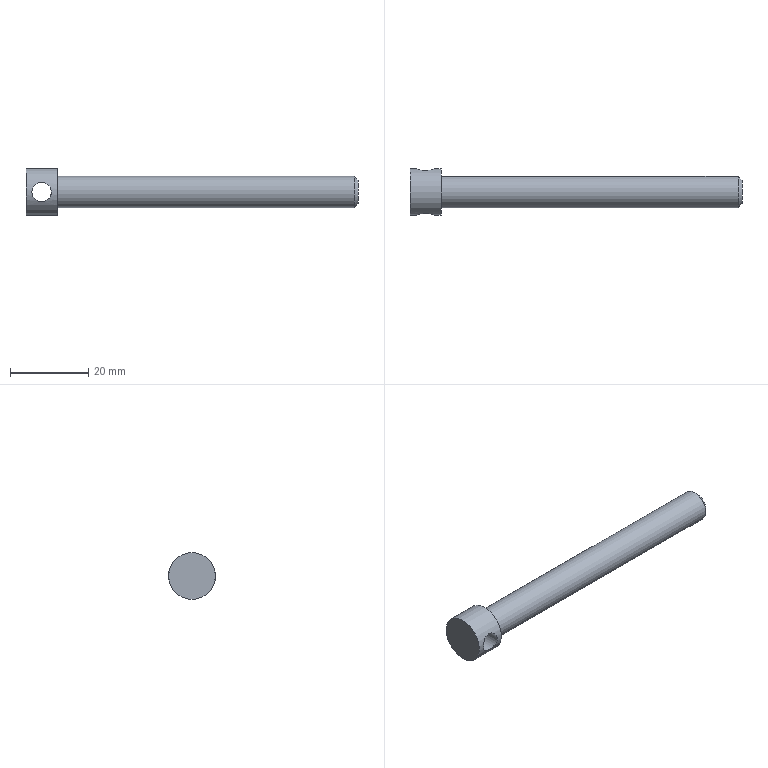Component | NX | TORQUE_SHAFT | 1 solid | 7 faces | box 85 x 12 x 12 mm | volume 4533 mm3 | cylinder 3 | plane 3 | cone 1 | commonest cylinder face diameters 12 x1 8 x1 5 x1
STEP:
#1=CARTESIAN_POINT('',(0.,0.,0.));
#2=DIRECTION('',(0.,0.,1.));
#3=DIRECTION('',(1.,0.,0.));
#4=AXIS2_PLACEMENT_3D('',#1,#2,#3);
#5=CARTESIAN_POINT('',(-16.764,70.391,12.));
#6=VERTEX_POINT('',#5);
#7=CARTESIAN_POINT('',(-16.764,70.391,18.));
#8=DIRECTION('',(-1.,0.,0.));
#9=DIRECTION('',(0.,0.,-1.));
#10=AXIS2_PLACEMENT_3D('',#7,#8,#9);
#11=CIRCLE('',#10,6.);
#12=CARTESIAN_POINT('',(-24.764,70.391,18.));
#13=DIRECTION('',(1.,0.,0.));
#14=DIRECTION('',(0.,0.,-1.));
#15=AXIS2_PLACEMENT_3D('',#12,#13,#14);
#16=CYLINDRICAL_SURFACE('',#15,6.);
#17=CARTESIAN_POINT('',(6.283,8.));
#18=DIRECTION('',(-1.,0.));
#19=VECTOR('',#18,1.);
#20=LINE('',#17,#19);
#21=(GEOMETRIC_REPRESENTATION_CONTEXT(2)PARAMETRIC_REPRESENTATION_CONTEXT()REPRESENTATION_CONTEXT('',''));
#22=DEFINITIONAL_REPRESENTATION('',(#20),#21);
#23=PCURVE('',#16,#22);
#24=CARTESIAN_POINT('',(-16.764,70.391,18.));
#25=DIRECTION('',(1.,0.,0.));
#26=DIRECTION('',(0.,0.,-1.));
#27=AXIS2_PLACEMENT_3D('',#24,#25,#26);
#28=PLANE('',#27);
#29=CARTESIAN_POINT('',(6.,0.));
#30=CARTESIAN_POINT('',(6.,-10.392));
#31=CARTESIAN_POINT('',(-3.,-5.196));
#32=CARTESIAN_POINT('',(-12.,-0.));
#33=CARTESIAN_POINT('',(-3.,5.196));
#34=CARTESIAN_POINT('',(6.,10.392));
#35=CARTESIAN_POINT('',(6.,0.));
#36=(BOUNDED_CURVE()B_SPLINE_CURVE(2,(#29,#30,#31,#32,#33,#34,#35),.UNSPECIFIED.,.T.,.F.)B_SPLINE_CURVE_WITH_KNOTS((1,2,2,2,2,1),(-2.094,0.,2.094,4.189,6.283,8.378),.UNSPECIFIED.)CURVE()GEOMETRIC_REPRESENTATION_ITEM()RATIONAL_B_SPLINE_CURVE((1.,0.5,1.,0.5,1.,0.5,1.))REPRESENTATION_ITEM(''));
#37=(GEOMETRIC_REPRESENTATION_CONTEXT(2)PARAMETRIC_REPRESENTATION_CONTEXT()REPRESENTATION_CONTEXT('',''));
#38=DEFINITIONAL_REPRESENTATION('',(#36),#37);
#39=PCURVE('',#28,#38);
#40=SURFACE_CURVE('',#11,(#23,#39),.PCURVE_S1.);
#41=EDGE_CURVE('',#6,#6,#40,.T.);
#42=ORIENTED_EDGE('',*,*,#41,.T.);
#43=CARTESIAN_POINT('',(-24.764,70.391,12.));
#44=VERTEX_POINT('',#43);
#45=CARTESIAN_POINT('',(-24.764,70.391,12.));
#46=CARTESIAN_POINT('',(-16.764,70.391,12.));
#47=B_SPLINE_CURVE_WITH_KNOTS('',1,(#45,#46),.UNSPECIFIED.,.F.,.F.,(2,2),(0.,8.),.PIECEWISE_BEZIER_KNOTS.);
#48=CARTESIAN_POINT('',(0.,0.));
#49=DIRECTION('',(0.,1.));
#50=VECTOR('',#49,1.);
#51=LINE('',#48,#50);
#52=(GEOMETRIC_REPRESENTATION_CONTEXT(2)PARAMETRIC_REPRESENTATION_CONTEXT()REPRESENTATION_CONTEXT('',''));
#53=DEFINITIONAL_REPRESENTATION('',(#51),#52);
#54=PCURVE('',#16,#53);
#55=CARTESIAN_POINT('',(6.283,0.));
#56=DIRECTION('',(0.,1.));
#57=VECTOR('',#56,1.);
#58=LINE('',#55,#57);
#59=(GEOMETRIC_REPRESENTATION_CONTEXT(2)PARAMETRIC_REPRESENTATION_CONTEXT()REPRESENTATION_CONTEXT('',''));
#60=DEFINITIONAL_REPRESENTATION('',(#58),#59);
#61=PCURVE('',#16,#60);
#62=SEAM_CURVE('',#47,(#54,#61),.PCURVE_S1.);
#63=EDGE_CURVE('',#44,#6,#62,.T.);
#64=ORIENTED_EDGE('',*,*,#63,.F.);
#65=CARTESIAN_POINT('',(-24.764,70.391,18.));
#66=DIRECTION('',(1.,0.,0.));
#67=DIRECTION('',(0.,0.,-1.));
#68=AXIS2_PLACEMENT_3D('',#65,#66,#67);
#69=CIRCLE('',#68,6.);
#70=CARTESIAN_POINT('',(0.,0.));
#71=DIRECTION('',(1.,0.));
#72=VECTOR('',#71,1.);
#73=LINE('',#70,#72);
#74=(GEOMETRIC_REPRESENTATION_CONTEXT(2)PARAMETRIC_REPRESENTATION_CONTEXT()REPRESENTATION_CONTEXT('',''));
#75=DEFINITIONAL_REPRESENTATION('',(#73),#74);
#76=PCURVE('',#16,#75);
#77=CARTESIAN_POINT('',(-24.764,70.391,18.));
#78=DIRECTION('',(-1.,0.,0.));
#79=DIRECTION('',(0.,0.,1.));
#80=AXIS2_PLACEMENT_3D('',#77,#78,#79);
#81=PLANE('',#80);
#82=CARTESIAN_POINT('',(-6.,0.));
#83=CARTESIAN_POINT('',(-6.,10.392));
#84=CARTESIAN_POINT('',(3.,5.196));
#85=CARTESIAN_POINT('',(12.,0.));
#86=CARTESIAN_POINT('',(3.,-5.196));
#87=CARTESIAN_POINT('',(-6.,-10.392));
#88=CARTESIAN_POINT('',(-6.,0.));
#89=(BOUNDED_CURVE()B_SPLINE_CURVE(2,(#82,#83,#84,#85,#86,#87,#88),.UNSPECIFIED.,.T.,.F.)B_SPLINE_CURVE_WITH_KNOTS((1,2,2,2,2,1),(-2.094,0.,2.094,4.189,6.283,8.378),.UNSPECIFIED.)CURVE()GEOMETRIC_REPRESENTATION_ITEM()RATIONAL_B_SPLINE_CURVE((1.,0.5,1.,0.5,1.,0.5,1.))REPRESENTATION_ITEM(''));
#90=(GEOMETRIC_REPRESENTATION_CONTEXT(2)PARAMETRIC_REPRESENTATION_CONTEXT()REPRESENTATION_CONTEXT('',''));
#91=DEFINITIONAL_REPRESENTATION('',(#89),#90);
#92=PCURVE('',#81,#91);
#93=SURFACE_CURVE('',#69,(#76,#92),.PCURVE_S1.);
#94=EDGE_CURVE('',#44,#44,#93,.T.);
#95=ORIENTED_EDGE('',*,*,#94,.T.);
#96=ORIENTED_EDGE('',*,*,#63,.T.);
#97=EDGE_LOOP('',(#42,#64,#95,#96));
#98=FACE_BOUND('',#97,.T.);
#99=CARTESIAN_POINT('',(-18.264,76.391,18.));
#100=VERTEX_POINT('',#99);
#101=CARTESIAN_POINT('',(-18.264,76.391,18.));
#102=CARTESIAN_POINT('',(-18.264,76.391,18.267));
#103=CARTESIAN_POINT('',(-18.308,76.373,18.538));
#104=CARTESIAN_POINT('',(-18.392,76.339,18.789));
#105=CARTESIAN_POINT('',(-18.475,76.306,19.04));
#106=CARTESIAN_POINT('',(-18.6,76.258,19.279));
#107=CARTESIAN_POINT('',(-18.755,76.204,19.489));
#108=CARTESIAN_POINT('',(-18.918,76.148,19.708));
#109=CARTESIAN_POINT('',(-19.119,76.084,19.902));
#110=CARTESIAN_POINT('',(-19.343,76.028,20.057));
#111=CARTESIAN_POINT('',(-19.579,75.968,20.22));
#112=CARTESIAN_POINT('',(-19.848,75.915,20.345));
#113=CARTESIAN_POINT('',(-20.13,75.883,20.418));
#114=CARTESIAN_POINT('',(-20.397,75.852,20.488));
#115=CARTESIAN_POINT('',(-20.683,75.839,20.514));
#116=CARTESIAN_POINT('',(-20.96,75.849,20.492));
#117=CARTESIAN_POINT('',(-21.216,75.859,20.472));
#118=CARTESIAN_POINT('',(-21.471,75.887,20.411));
#119=CARTESIAN_POINT('',(-21.706,75.927,20.316));
#120=CARTESIAN_POINT('',(-21.947,75.968,20.218));
#121=CARTESIAN_POINT('',(-22.172,76.021,20.081));
#122=CARTESIAN_POINT('',(-22.369,76.077,19.917));
#123=CARTESIAN_POINT('',(-22.582,76.137,19.738));
#124=CARTESIAN_POINT('',(-22.768,76.201,19.521));
#125=CARTESIAN_POINT('',(-22.911,76.253,19.28));
#126=CARTESIAN_POINT('',(-23.057,76.307,19.035));
#127=CARTESIAN_POINT('',(-23.164,76.35,18.757));
#128=CARTESIAN_POINT('',(-23.219,76.373,18.472));
#129=CARTESIAN_POINT('',(-23.27,76.394,18.205));
#130=CARTESIAN_POINT('',(-23.277,76.397,17.924));
#131=CARTESIAN_POINT('',(-23.24,76.381,17.655));
#132=CARTESIAN_POINT('',(-23.204,76.367,17.398));
#133=CARTESIAN_POINT('',(-23.127,76.335,17.145));
#134=CARTESIAN_POINT('',(-23.016,76.293,16.915));
#135=CARTESIAN_POINT('',(-22.902,76.249,16.677));
#136=CARTESIAN_POINT('',(-22.748,76.193,16.457));
#137=CARTESIAN_POINT('',(-22.567,76.136,16.269));
#138=CARTESIAN_POINT('',(-22.373,76.075,16.067));
#139=CARTESIAN_POINT('',(-22.142,76.012,15.896));
#140=CARTESIAN_POINT('',(-21.891,75.961,15.768));
#141=CARTESIAN_POINT('',(-21.636,75.909,15.64));
#142=CARTESIAN_POINT('',(-21.351,75.87,15.553));
#143=CARTESIAN_POINT('',(-21.064,75.854,15.518));
#144=CARTESIAN_POINT('',(-20.798,75.839,15.486));
#145=CARTESIAN_POINT('',(-20.522,75.845,15.497));
#146=CARTESIAN_POINT('',(-20.261,75.869,15.551));
#147=CARTESIAN_POINT('',(-20.011,75.892,15.602));
#148=CARTESIAN_POINT('',(-19.769,75.932,15.693));
#149=CARTESIAN_POINT('',(-19.549,75.979,15.815));
#150=CARTESIAN_POINT('',(-19.316,76.03,15.944));
#151=CARTESIAN_POINT('',(-19.104,76.09,16.112));
#152=CARTESIAN_POINT('',(-18.924,76.148,16.307));
#153=CARTESIAN_POINT('',(-18.732,76.209,16.516));
#154=CARTESIAN_POINT('',(-18.572,76.269,16.763));
#155=CARTESIAN_POINT('',(-18.461,76.312,17.028));
#156=CARTESIAN_POINT('',(-18.351,76.355,17.288));
#157=CARTESIAN_POINT('',(-18.284,76.383,17.573));
#158=CARTESIAN_POINT('',(-18.268,76.39,17.858));
#159=CARTESIAN_POINT('',(-18.265,76.391,17.906));
#160=CARTESIAN_POINT('',(-18.264,76.391,17.953));
#161=CARTESIAN_POINT('',(-18.264,76.391,18.));
#162=B_SPLINE_CURVE_WITH_KNOTS('',3,(#101,#102,#103,#104,#105,#106,#107,#108,#109,#110,#111,#112,#113,#114,#115,#116,#117,#118,#119,#120,#121,#122,#123,#124,#125,#126,#127,#128,#129,#130,#131,#132,#133,#134,#135,#136,#137,#138,#139,#140,#141,#142,#143,#144,#145,#146,#147,#148,#149,#150,#151,#152,#153,#154,#155,#156,#157,#158,#159,#160,#161),.UNSPECIFIED.,.T.,.F.,(1,3,3,3,3,3,3,3,3,3,3,3,3,3,3,3,3,3,3,3,3,3,1),(-0.008825,0.,0.05069,0.1012,0.1541,0.2097,0.2625,0.3112,0.3609,0.4149,0.4703,0.522,0.5711,0.6217,0.6761,0.7313,0.7821,0.8305,0.8818,0.937,0.9912,1.,1.051),.UNSPECIFIED.);
#163=CARTESIAN_POINT('',(1.571,6.5));
#164=CARTESIAN_POINT('',(1.581,6.5));
#165=CARTESIAN_POINT('',(1.601,6.496));
#166=CARTESIAN_POINT('',(1.631,6.476));
#167=CARTESIAN_POINT('',(1.66,6.444));
#168=CARTESIAN_POINT('',(1.69,6.399));
#169=CARTESIAN_POINT('',(1.718,6.342));
#170=CARTESIAN_POINT('',(1.746,6.273));
#171=CARTESIAN_POINT('',(1.773,6.192));
#172=CARTESIAN_POINT('',(1.799,6.101));
#173=CARTESIAN_POINT('',(1.824,6.));
#174=CARTESIAN_POINT('',(1.848,5.889));
#175=CARTESIAN_POINT('',(1.87,5.769));
#176=CARTESIAN_POINT('',(1.891,5.639));
#177=CARTESIAN_POINT('',(1.911,5.502));
#178=CARTESIAN_POINT('',(1.929,5.357));
#179=CARTESIAN_POINT('',(1.945,5.205));
#180=CARTESIAN_POINT('',(1.959,5.046));
#181=CARTESIAN_POINT('',(1.972,4.881));
#182=CARTESIAN_POINT('',(1.982,4.712));
#183=CARTESIAN_POINT('',(1.99,4.539));
#184=CARTESIAN_POINT('',(1.996,4.362));
#185=CARTESIAN_POINT('',(2.,4.182));
#186=CARTESIAN_POINT('',(2.001,4.002));
#187=CARTESIAN_POINT('',(2.,3.822));
#188=CARTESIAN_POINT('',(1.996,3.643));
#189=CARTESIAN_POINT('',(1.99,3.465));
#190=CARTESIAN_POINT('',(1.982,3.291));
#191=CARTESIAN_POINT('',(1.972,3.121));
#192=CARTESIAN_POINT('',(1.96,2.957));
#193=CARTESIAN_POINT('',(1.945,2.797));
#194=CARTESIAN_POINT('',(1.929,2.645));
#195=CARTESIAN_POINT('',(1.911,2.499));
#196=CARTESIAN_POINT('',(1.891,2.362));
#197=CARTESIAN_POINT('',(1.87,2.233));
#198=CARTESIAN_POINT('',(1.848,2.112));
#199=CARTESIAN_POINT('',(1.824,2.001));
#200=CARTESIAN_POINT('',(1.799,1.899));
#201=CARTESIAN_POINT('',(1.773,1.808));
#202=CARTESIAN_POINT('',(1.746,1.728));
#203=CARTESIAN_POINT('',(1.719,1.659));
#204=CARTESIAN_POINT('',(1.69,1.602));
#205=CARTESIAN_POINT('',(1.661,1.557));
#206=CARTESIAN_POINT('',(1.631,1.524));
#207=CARTESIAN_POINT('',(1.601,1.505));
#208=CARTESIAN_POINT('',(1.571,1.498));
#209=CARTESIAN_POINT('',(1.541,1.504));
#210=CARTESIAN_POINT('',(1.511,1.523));
#211=CARTESIAN_POINT('',(1.482,1.556));
#212=CARTESIAN_POINT('',(1.452,1.601));
#213=CARTESIAN_POINT('',(1.424,1.658));
#214=CARTESIAN_POINT('',(1.396,1.726));
#215=CARTESIAN_POINT('',(1.369,1.806));
#216=CARTESIAN_POINT('',(1.343,1.897));
#217=CARTESIAN_POINT('',(1.318,1.999));
#218=CARTESIAN_POINT('',(1.294,2.11));
#219=CARTESIAN_POINT('',(1.272,2.23));
#220=CARTESIAN_POINT('',(1.251,2.359));
#221=CARTESIAN_POINT('',(1.231,2.497));
#222=CARTESIAN_POINT('',(1.213,2.642));
#223=CARTESIAN_POINT('',(1.197,2.795));
#224=CARTESIAN_POINT('',(1.182,2.952));
#225=CARTESIAN_POINT('',(1.17,3.117));
#226=CARTESIAN_POINT('',(1.16,3.287));
#227=CARTESIAN_POINT('',(1.151,3.461));
#228=CARTESIAN_POINT('',(1.145,3.638));
#229=CARTESIAN_POINT('',(1.142,3.816));
#230=CARTESIAN_POINT('',(1.141,3.997));
#231=CARTESIAN_POINT('',(1.142,4.178));
#232=CARTESIAN_POINT('',(1.145,4.358));
#233=CARTESIAN_POINT('',(1.151,4.534));
#234=CARTESIAN_POINT('',(1.159,4.709));
#235=CARTESIAN_POINT('',(1.17,4.879));
#236=CARTESIAN_POINT('',(1.182,5.044));
#237=CARTESIAN_POINT('',(1.196,5.203));
#238=CARTESIAN_POINT('',(1.213,5.355));
#239=CARTESIAN_POINT('',(1.231,5.501));
#240=CARTESIAN_POINT('',(1.25,5.639));
#241=CARTESIAN_POINT('',(1.271,5.768));
#242=CARTESIAN_POINT('',(1.294,5.888));
#243=CARTESIAN_POINT('',(1.317,5.999));
#244=CARTESIAN_POINT('',(1.342,6.101));
#245=CARTESIAN_POINT('',(1.369,6.192));
#246=CARTESIAN_POINT('',(1.395,6.273));
#247=CARTESIAN_POINT('',(1.423,6.341));
#248=CARTESIAN_POINT('',(1.452,6.398));
#249=CARTESIAN_POINT('',(1.481,6.443));
#250=CARTESIAN_POINT('',(1.511,6.476));
#251=CARTESIAN_POINT('',(1.54,6.496));
#252=CARTESIAN_POINT('',(1.561,6.5));
#253=CARTESIAN_POINT('',(1.571,6.5));
#254=B_SPLINE_CURVE_WITH_KNOTS('',3,(#163,#164,#165,#166,#167,#168,#169,#170,#171,#172,#173,#174,#175,#176,#177,#178,#179,#180,#181,#182,#183,#184,#185,#186,#187,#188,#189,#190,#191,#192,#193,#194,#195,#196,#197,#198,#199,#200,#201,#202,#203,#204,#205,#206,#207,#208,#209,#210,#211,#212,#213,#214,#215,#216,#217,#218,#219,#220,#221,#222,#223,#224,#225,#226,#227,#228,#229,#230,#231,#232,#233,#234,#235,#236,#237,#238,#239,#240,#241,#242,#243,#244,#245,#246,#247,#248,#249,#250,#251,#252,#253),.UNSPECIFIED.,.T.,.F.,(4,1,1,1,1,1,1,1,1,1,1,1,1,1,1,1,1,1,1,1,1,1,1,1,1,1,1,1,1,1,1,1,1,1,1,1,1,1,1,1,1,1,1,1,1,1,1,1,1,1,1,1,1,1,1,1,1,1,1,1,1,1,1,1,1,1,1,1,1,1,1,1,1,1,1,1,1,1,1,1,1,1,1,1,1,1,1,1,4),(0.,0.01136,0.02273,0.03409,0.04545,0.05682,0.06818,0.07955,0.09091,0.1023,0.1136,0.125,0.1364,0.1477,0.1591,0.1705,0.1818,0.1932,0.2045,0.2159,0.2273,0.2386,0.25,0.2614,0.2727,0.2841,0.2955,0.3068,0.3182,0.3295,0.3409,0.3523,0.3636,0.375,0.3864,0.3977,0.4091,0.4205,0.4318,0.4432,0.4545,0.4659,0.4773,0.4886,0.5,0.5114,0.5227,0.5341,0.5455,0.5568,0.5682,0.5795,0.5909,0.6023,0.6136,0.625,0.6364,0.6477,0.6591,0.6705,0.6818,0.6932,0.7045,0.7159,0.7273,0.7386,0.75,0.7614,0.7727,0.7841,0.7955,0.8068,0.8182,0.8295,0.8409,0.8523,0.8636,0.875,0.8864,0.8977,0.9091,0.9205,0.9318,0.9432,0.9545,0.9659,0.9773,0.9886,1.),.QUASI_UNIFORM_KNOTS.);
#255=(GEOMETRIC_REPRESENTATION_CONTEXT(2)PARAMETRIC_REPRESENTATION_CONTEXT()REPRESENTATION_CONTEXT('',''));
#256=DEFINITIONAL_REPRESENTATION('',(#254),#255);
#257=PCURVE('',#16,#256);
#258=CARTESIAN_POINT('',(-20.764,62.391,18.));
#259=DIRECTION('',(0.,1.,0.));
#260=DIRECTION('',(1.,0.,0.));
#261=AXIS2_PLACEMENT_3D('',#258,#259,#260);
#262=CYLINDRICAL_SURFACE('',#261,2.5);
#263=CARTESIAN_POINT('',(6.283,14.));
#264=CARTESIAN_POINT('',(6.259,14.));
#265=CARTESIAN_POINT('',(6.211,13.998));
#266=CARTESIAN_POINT('',(6.139,13.99));
#267=CARTESIAN_POINT('',(6.067,13.977));
#268=CARTESIAN_POINT('',(5.995,13.958));
#269=CARTESIAN_POINT('',(5.923,13.936));
#270=CARTESIAN_POINT('',(5.852,13.909));
#271=CARTESIAN_POINT('',(5.781,13.878));
#272=CARTESIAN_POINT('',(5.709,13.845));
#273=CARTESIAN_POINT('',(5.639,13.809));
#274=CARTESIAN_POINT('',(5.568,13.772));
#275=CARTESIAN_POINT('',(5.498,13.734));
#276=CARTESIAN_POINT('',(5.427,13.695));
#277=CARTESIAN_POINT('',(5.356,13.657));
#278=CARTESIAN_POINT('',(5.286,13.62));
#279=CARTESIAN_POINT('',(5.215,13.585));
#280=CARTESIAN_POINT('',(5.144,13.553));
#281=CARTESIAN_POINT('',(5.072,13.524));
#282=CARTESIAN_POINT('',(5.001,13.5));
#283=CARTESIAN_POINT('',(4.93,13.48));
#284=CARTESIAN_POINT('',(4.858,13.466));
#285=CARTESIAN_POINT('',(4.785,13.457));
#286=CARTESIAN_POINT('',(4.713,13.454));
#287=CARTESIAN_POINT('',(4.641,13.456));
#288=CARTESIAN_POINT('',(4.569,13.465));
#289=CARTESIAN_POINT('',(4.497,13.48));
#290=CARTESIAN_POINT('',(4.425,13.5));
#291=CARTESIAN_POINT('',(4.353,13.524));
#292=CARTESIAN_POINT('',(4.282,13.553));
#293=CARTESIAN_POINT('',(4.211,13.585));
#294=CARTESIAN_POINT('',(4.14,13.62));
#295=CARTESIAN_POINT('',(4.069,13.657));
#296=CARTESIAN_POINT('',(3.999,13.695));
#297=CARTESIAN_POINT('',(3.928,13.733));
#298=CARTESIAN_POINT('',(3.857,13.772));
#299=CARTESIAN_POINT('',(3.786,13.809));
#300=CARTESIAN_POINT('',(3.716,13.845));
#301=CARTESIAN_POINT('',(3.645,13.878));
#302=CARTESIAN_POINT('',(3.574,13.908));
#303=CARTESIAN_POINT('',(3.502,13.935));
#304=CARTESIAN_POINT('',(3.431,13.958));
#305=CARTESIAN_POINT('',(3.359,13.977));
#306=CARTESIAN_POINT('',(3.287,13.99));
#307=CARTESIAN_POINT('',(3.215,13.998));
#308=CARTESIAN_POINT('',(3.143,14.001));
#309=CARTESIAN_POINT('',(3.07,13.998));
#310=CARTESIAN_POINT('',(2.998,13.99));
#311=CARTESIAN_POINT('',(2.926,13.977));
#312=CARTESIAN_POINT('',(2.854,13.959));
#313=CARTESIAN_POINT('',(2.782,13.936));
#314=CARTESIAN_POINT('',(2.711,13.909));
#315=CARTESIAN_POINT('',(2.64,13.879));
#316=CARTESIAN_POINT('',(2.569,13.845));
#317=CARTESIAN_POINT('',(2.498,13.81));
#318=CARTESIAN_POINT('',(2.427,13.772));
#319=CARTESIAN_POINT('',(2.357,13.734));
#320=CARTESIAN_POINT('',(2.286,13.695));
#321=CARTESIAN_POINT('',(2.215,13.657));
#322=CARTESIAN_POINT('',(2.144,13.62));
#323=CARTESIAN_POINT('',(2.073,13.585));
#324=CARTESIAN_POINT('',(2.003,13.553));
#325=CARTESIAN_POINT('',(1.932,13.525));
#326=CARTESIAN_POINT('',(1.86,13.5));
#327=CARTESIAN_POINT('',(1.788,13.48));
#328=CARTESIAN_POINT('',(1.716,13.465));
#329=CARTESIAN_POINT('',(1.644,13.457));
#330=CARTESIAN_POINT('',(1.572,13.454));
#331=CARTESIAN_POINT('',(1.5,13.457));
#332=CARTESIAN_POINT('',(1.427,13.465));
#333=CARTESIAN_POINT('',(1.356,13.48));
#334=CARTESIAN_POINT('',(1.284,13.499));
#335=CARTESIAN_POINT('',(1.212,13.524));
#336=CARTESIAN_POINT('',(1.14,13.553));
#337=CARTESIAN_POINT('',(1.069,13.585));
#338=CARTESIAN_POINT('',(0.9984,13.62));
#339=CARTESIAN_POINT('',(0.9275,13.657));
#340=CARTESIAN_POINT('',(0.8566,13.695));
#341=CARTESIAN_POINT('',(0.7859,13.733));
#342=CARTESIAN_POINT('',(0.7156,13.772));
#343=CARTESIAN_POINT('',(0.6449,13.809));
#344=CARTESIAN_POINT('',(0.5739,13.845));
#345=CARTESIAN_POINT('',(0.5028,13.878));
#346=CARTESIAN_POINT('',(0.4316,13.909));
#347=CARTESIAN_POINT('',(0.3606,13.935));
#348=CARTESIAN_POINT('',(0.2889,13.958));
#349=CARTESIAN_POINT('',(0.2169,13.976));
#350=CARTESIAN_POINT('',(0.1446,13.99));
#351=CARTESIAN_POINT('',(0.07286,13.998));
#352=CARTESIAN_POINT('',(0.02446,14.));
#353=CARTESIAN_POINT('',(-0.,14.));
#354=B_SPLINE_CURVE_WITH_KNOTS('',3,(#263,#264,#265,#266,#267,#268,#269,#270,#271,#272,#273,#274,#275,#276,#277,#278,#279,#280,#281,#282,#283,#284,#285,#286,#287,#288,#289,#290,#291,#292,#293,#294,#295,#296,#297,#298,#299,#300,#301,#302,#303,#304,#305,#306,#307,#308,#309,#310,#311,#312,#313,#314,#315,#316,#317,#318,#319,#320,#321,#322,#323,#324,#325,#326,#327,#328,#329,#330,#331,#332,#333,#334,#335,#336,#337,#338,#339,#340,#341,#342,#343,#344,#345,#346,#347,#348,#349,#350,#351,#352,#353),.UNSPECIFIED.,.F.,.F.,(4,1,1,1,1,1,1,1,1,1,1,1,1,1,1,1,1,1,1,1,1,1,1,1,1,1,1,1,1,1,1,1,1,1,1,1,1,1,1,1,1,1,1,1,1,1,1,1,1,1,1,1,1,1,1,1,1,1,1,1,1,1,1,1,1,1,1,1,1,1,1,1,1,1,1,1,1,1,1,1,1,1,1,1,1,1,1,1,4),(0.,0.01136,0.02273,0.03409,0.04545,0.05682,0.06818,0.07955,0.09091,0.1023,0.1136,0.125,0.1364,0.1477,0.1591,0.1705,0.1818,0.1932,0.2045,0.2159,0.2273,0.2386,0.25,0.2614,0.2727,0.2841,0.2955,0.3068,0.3182,0.3295,0.3409,0.3523,0.3636,0.375,0.3864,0.3977,0.4091,0.4205,0.4318,0.4432,0.4545,0.4659,0.4773,0.4886,0.5,0.5114,0.5227,0.5341,0.5455,0.5568,0.5682,0.5795,0.5909,0.6023,0.6136,0.625,0.6364,0.6477,0.6591,0.6705,0.6818,0.6932,0.7045,0.7159,0.7273,0.7386,0.75,0.7614,0.7727,0.7841,0.7955,0.8068,0.8182,0.8295,0.8409,0.8523,0.8636,0.875,0.8864,0.8977,0.9091,0.9205,0.9318,0.9432,0.9545,0.9659,0.9773,0.9886,1.),.QUASI_UNIFORM_KNOTS.);
#355=(GEOMETRIC_REPRESENTATION_CONTEXT(2)PARAMETRIC_REPRESENTATION_CONTEXT()REPRESENTATION_CONTEXT('',''));
#356=DEFINITIONAL_REPRESENTATION('',(#354),#355);
#357=PCURVE('',#262,#356);
#358=SURFACE_CURVE('',#162,(#257,#357),.PCURVE_S1.);
#359=EDGE_CURVE('',#100,#100,#358,.T.);
#360=ORIENTED_EDGE('',*,*,#359,.T.);
#361=EDGE_LOOP('',(#360));
#362=FACE_BOUND('',#361,.T.);
#363=CARTESIAN_POINT('',(-18.264,64.391,18.));
#364=VERTEX_POINT('',#363);
#365=CARTESIAN_POINT('',(-18.264,64.391,18.));
#366=CARTESIAN_POINT('',(-18.264,64.391,17.733));
#367=CARTESIAN_POINT('',(-18.308,64.41,17.462));
#368=CARTESIAN_POINT('',(-18.392,64.444,17.211));
#369=CARTESIAN_POINT('',(-18.475,64.477,16.96));
#370=CARTESIAN_POINT('',(-18.6,64.525,16.721));
#371=CARTESIAN_POINT('',(-18.755,64.579,16.511));
#372=CARTESIAN_POINT('',(-18.918,64.635,16.292));
#373=CARTESIAN_POINT('',(-19.119,64.699,16.098));
#374=CARTESIAN_POINT('',(-19.343,64.755,15.943));
#375=CARTESIAN_POINT('',(-19.579,64.815,15.78));
#376=CARTESIAN_POINT('',(-19.848,64.868,15.655));
#377=CARTESIAN_POINT('',(-20.13,64.9,15.582));
#378=CARTESIAN_POINT('',(-20.397,64.931,15.512));
#379=CARTESIAN_POINT('',(-20.683,64.944,15.486));
#380=CARTESIAN_POINT('',(-20.96,64.934,15.508));
#381=CARTESIAN_POINT('',(-21.216,64.924,15.528));
#382=CARTESIAN_POINT('',(-21.471,64.896,15.589));
#383=CARTESIAN_POINT('',(-21.706,64.856,15.684));
#384=CARTESIAN_POINT('',(-21.947,64.815,15.782));
#385=CARTESIAN_POINT('',(-22.172,64.761,15.919));
#386=CARTESIAN_POINT('',(-22.369,64.706,16.083));
#387=CARTESIAN_POINT('',(-22.582,64.646,16.262));
#388=CARTESIAN_POINT('',(-22.768,64.582,16.479));
#389=CARTESIAN_POINT('',(-22.911,64.53,16.72));
#390=CARTESIAN_POINT('',(-23.057,64.476,16.965));
#391=CARTESIAN_POINT('',(-23.164,64.433,17.243));
#392=CARTESIAN_POINT('',(-23.219,64.41,17.528));
#393=CARTESIAN_POINT('',(-23.27,64.389,17.795));
#394=CARTESIAN_POINT('',(-23.277,64.386,18.076));
#395=CARTESIAN_POINT('',(-23.24,64.401,18.345));
#396=CARTESIAN_POINT('',(-23.204,64.416,18.602));
#397=CARTESIAN_POINT('',(-23.127,64.448,18.855));
#398=CARTESIAN_POINT('',(-23.016,64.49,19.085));
#399=CARTESIAN_POINT('',(-22.902,64.534,19.323));
#400=CARTESIAN_POINT('',(-22.748,64.59,19.543));
#401=CARTESIAN_POINT('',(-22.567,64.647,19.731));
#402=CARTESIAN_POINT('',(-22.373,64.707,19.933));
#403=CARTESIAN_POINT('',(-22.142,64.771,20.104));
#404=CARTESIAN_POINT('',(-21.891,64.822,20.232));
#405=CARTESIAN_POINT('',(-21.636,64.873,20.36));
#406=CARTESIAN_POINT('',(-21.351,64.913,20.447));
#407=CARTESIAN_POINT('',(-21.064,64.929,20.482));
#408=CARTESIAN_POINT('',(-20.798,64.943,20.514));
#409=CARTESIAN_POINT('',(-20.522,64.938,20.503));
#410=CARTESIAN_POINT('',(-20.261,64.914,20.449));
#411=CARTESIAN_POINT('',(-20.011,64.891,20.398));
#412=CARTESIAN_POINT('',(-19.769,64.851,20.307));
#413=CARTESIAN_POINT('',(-19.549,64.803,20.185));
#414=CARTESIAN_POINT('',(-19.316,64.753,20.056));
#415=CARTESIAN_POINT('',(-19.104,64.693,19.888));
#416=CARTESIAN_POINT('',(-18.924,64.635,19.693));
#417=CARTESIAN_POINT('',(-18.732,64.574,19.484));
#418=CARTESIAN_POINT('',(-18.572,64.514,19.237));
#419=CARTESIAN_POINT('',(-18.461,64.471,18.972));
#420=CARTESIAN_POINT('',(-18.351,64.428,18.712));
#421=CARTESIAN_POINT('',(-18.284,64.4,18.427));
#422=CARTESIAN_POINT('',(-18.268,64.393,18.142));
#423=CARTESIAN_POINT('',(-18.265,64.392,18.094));
#424=CARTESIAN_POINT('',(-18.264,64.391,18.047));
#425=CARTESIAN_POINT('',(-18.264,64.391,18.));
#426=B_SPLINE_CURVE_WITH_KNOTS('',3,(#365,#366,#367,#368,#369,#370,#371,#372,#373,#374,#375,#376,#377,#378,#379,#380,#381,#382,#383,#384,#385,#386,#387,#388,#389,#390,#391,#392,#393,#394,#395,#396,#397,#398,#399,#400,#401,#402,#403,#404,#405,#406,#407,#408,#409,#410,#411,#412,#413,#414,#415,#416,#417,#418,#419,#420,#421,#422,#423,#424,#425),.UNSPECIFIED.,.T.,.F.,(1,3,3,3,3,3,3,3,3,3,3,3,3,3,3,3,3,3,3,3,3,3,1),(-0.008825,0.,0.05069,0.1012,0.1541,0.2097,0.2625,0.3112,0.3609,0.4149,0.4703,0.522,0.5711,0.6217,0.6761,0.7313,0.7821,0.8305,0.8818,0.937,0.9912,1.,1.051),.UNSPECIFIED.);
#427=CARTESIAN_POINT('',(4.712,6.5));
#428=CARTESIAN_POINT('',(4.722,6.5));
#429=CARTESIAN_POINT('',(4.742,6.496));
#430=CARTESIAN_POINT('',(4.772,6.476));
#431=CARTESIAN_POINT('',(4.802,6.444));
#432=CARTESIAN_POINT('',(4.831,6.399));
#433=CARTESIAN_POINT('',(4.86,6.342));
#434=CARTESIAN_POINT('',(4.888,6.273));
#435=CARTESIAN_POINT('',(4.915,6.192));
#436=CARTESIAN_POINT('',(4.941,6.101));
#437=CARTESIAN_POINT('',(4.966,6.));
#438=CARTESIAN_POINT('',(4.989,5.889));
#439=CARTESIAN_POINT('',(5.012,5.769));
#440=CARTESIAN_POINT('',(5.033,5.639));
#441=CARTESIAN_POINT('',(5.052,5.502));
#442=CARTESIAN_POINT('',(5.07,5.357));
#443=CARTESIAN_POINT('',(5.086,5.205));
#444=CARTESIAN_POINT('',(5.101,5.046));
#445=CARTESIAN_POINT('',(5.113,4.881));
#446=CARTESIAN_POINT('',(5.124,4.712));
#447=CARTESIAN_POINT('',(5.132,4.539));
#448=CARTESIAN_POINT('',(5.138,4.362));
#449=CARTESIAN_POINT('',(5.141,4.182));
#450=CARTESIAN_POINT('',(5.143,4.002));
#451=CARTESIAN_POINT('',(5.141,3.822));
#452=CARTESIAN_POINT('',(5.138,3.643));
#453=CARTESIAN_POINT('',(5.132,3.465));
#454=CARTESIAN_POINT('',(5.124,3.291));
#455=CARTESIAN_POINT('',(5.113,3.121));
#456=CARTESIAN_POINT('',(5.101,2.957));
#457=CARTESIAN_POINT('',(5.087,2.797));
#458=CARTESIAN_POINT('',(5.07,2.645));
#459=CARTESIAN_POINT('',(5.053,2.499));
#460=CARTESIAN_POINT('',(5.033,2.362));
#461=CARTESIAN_POINT('',(5.012,2.233));
#462=CARTESIAN_POINT('',(4.99,2.112));
#463=CARTESIAN_POINT('',(4.966,2.001));
#464=CARTESIAN_POINT('',(4.941,1.899));
#465=CARTESIAN_POINT('',(4.915,1.808));
#466=CARTESIAN_POINT('',(4.888,1.728));
#467=CARTESIAN_POINT('',(4.86,1.659));
#468=CARTESIAN_POINT('',(4.832,1.602));
#469=CARTESIAN_POINT('',(4.802,1.557));
#470=CARTESIAN_POINT('',(4.773,1.524));
#471=CARTESIAN_POINT('',(4.743,1.505));
#472=CARTESIAN_POINT('',(4.713,1.498));
#473=CARTESIAN_POINT('',(4.683,1.504));
#474=CARTESIAN_POINT('',(4.653,1.523));
#475=CARTESIAN_POINT('',(4.623,1.556));
#476=CARTESIAN_POINT('',(4.594,1.601));
#477=CARTESIAN_POINT('',(4.565,1.658));
#478=CARTESIAN_POINT('',(4.537,1.726));
#479=CARTESIAN_POINT('',(4.511,1.806));
#480=CARTESIAN_POINT('',(4.484,1.897));
#481=CARTESIAN_POINT('',(4.459,1.999));
#482=CARTESIAN_POINT('',(4.436,2.11));
#483=CARTESIAN_POINT('',(4.413,2.23));
#484=CARTESIAN_POINT('',(4.392,2.359));
#485=CARTESIAN_POINT('',(4.373,2.497));
#486=CARTESIAN_POINT('',(4.355,2.642));
#487=CARTESIAN_POINT('',(4.338,2.795));
#488=CARTESIAN_POINT('',(4.324,2.952));
#489=CARTESIAN_POINT('',(4.312,3.117));
#490=CARTESIAN_POINT('',(4.301,3.287));
#491=CARTESIAN_POINT('',(4.293,3.461));
#492=CARTESIAN_POINT('',(4.287,3.638));
#493=CARTESIAN_POINT('',(4.283,3.816));
#494=CARTESIAN_POINT('',(4.282,3.997));
#495=CARTESIAN_POINT('',(4.283,4.178));
#496=CARTESIAN_POINT('',(4.287,4.358));
#497=CARTESIAN_POINT('',(4.293,4.534));
#498=CARTESIAN_POINT('',(4.301,4.709));
#499=CARTESIAN_POINT('',(4.311,4.879));
#500=CARTESIAN_POINT('',(4.324,5.044));
#501=CARTESIAN_POINT('',(4.338,5.203));
#502=CARTESIAN_POINT('',(4.354,5.355));
#503=CARTESIAN_POINT('',(4.372,5.501));
#504=CARTESIAN_POINT('',(4.392,5.639));
#505=CARTESIAN_POINT('',(4.413,5.768));
#506=CARTESIAN_POINT('',(4.435,5.888));
#507=CARTESIAN_POINT('',(4.459,5.999));
#508=CARTESIAN_POINT('',(4.484,6.101));
#509=CARTESIAN_POINT('',(4.51,6.192));
#510=CARTESIAN_POINT('',(4.537,6.273));
#511=CARTESIAN_POINT('',(4.565,6.341));
#512=CARTESIAN_POINT('',(4.593,6.398));
#513=CARTESIAN_POINT('',(4.623,6.443));
#514=CARTESIAN_POINT('',(4.652,6.476));
#515=CARTESIAN_POINT('',(4.682,6.496));
#516=CARTESIAN_POINT('',(4.702,6.5));
#517=CARTESIAN_POINT('',(4.712,6.5));
#518=B_SPLINE_CURVE_WITH_KNOTS('',3,(#427,#428,#429,#430,#431,#432,#433,#434,#435,#436,#437,#438,#439,#440,#441,#442,#443,#444,#445,#446,#447,#448,#449,#450,#451,#452,#453,#454,#455,#456,#457,#458,#459,#460,#461,#462,#463,#464,#465,#466,#467,#468,#469,#470,#471,#472,#473,#474,#475,#476,#477,#478,#479,#480,#481,#482,#483,#484,#485,#486,#487,#488,#489,#490,#491,#492,#493,#494,#495,#496,#497,#498,#499,#500,#501,#502,#503,#504,#505,#506,#507,#508,#509,#510,#511,#512,#513,#514,#515,#516,#517),.UNSPECIFIED.,.T.,.F.,(4,1,1,1,1,1,1,1,1,1,1,1,1,1,1,1,1,1,1,1,1,1,1,1,1,1,1,1,1,1,1,1,1,1,1,1,1,1,1,1,1,1,1,1,1,1,1,1,1,1,1,1,1,1,1,1,1,1,1,1,1,1,1,1,1,1,1,1,1,1,1,1,1,1,1,1,1,1,1,1,1,1,1,1,1,1,1,1,4),(0.,0.01136,0.02273,0.03409,0.04545,0.05682,0.06818,0.07955,0.09091,0.1023,0.1136,0.125,0.1364,0.1477,0.1591,0.1705,0.1818,0.1932,0.2045,0.2159,0.2273,0.2386,0.25,0.2614,0.2727,0.2841,0.2955,0.3068,0.3182,0.3295,0.3409,0.3523,0.3636,0.375,0.3864,0.3977,0.4091,0.4205,0.4318,0.4432,0.4545,0.4659,0.4773,0.4886,0.5,0.5114,0.5227,0.5341,0.5455,0.5568,0.5682,0.5795,0.5909,0.6023,0.6136,0.625,0.6364,0.6477,0.6591,0.6705,0.6818,0.6932,0.7045,0.7159,0.7273,0.7386,0.75,0.7614,0.7727,0.7841,0.7955,0.8068,0.8182,0.8295,0.8409,0.8523,0.8636,0.875,0.8864,0.8977,0.9091,0.9205,0.9318,0.9432,0.9545,0.9659,0.9773,0.9886,1.),.QUASI_UNIFORM_KNOTS.);
#519=(GEOMETRIC_REPRESENTATION_CONTEXT(2)PARAMETRIC_REPRESENTATION_CONTEXT()REPRESENTATION_CONTEXT('',''));
#520=DEFINITIONAL_REPRESENTATION('',(#518),#519);
#521=PCURVE('',#16,#520);
#522=CARTESIAN_POINT('',(0.,2.));
#523=CARTESIAN_POINT('',(0.02395,2.));
#524=CARTESIAN_POINT('',(0.07201,2.002));
#525=CARTESIAN_POINT('',(0.1443,2.01));
#526=CARTESIAN_POINT('',(0.2165,2.023));
#527=CARTESIAN_POINT('',(0.2884,2.042));
#528=CARTESIAN_POINT('',(0.3597,2.064));
#529=CARTESIAN_POINT('',(0.4312,2.091));
#530=CARTESIAN_POINT('',(0.5026,2.122));
#531=CARTESIAN_POINT('',(0.5738,2.155));
#532=CARTESIAN_POINT('',(0.6444,2.191));
#533=CARTESIAN_POINT('',(0.7149,2.228));
#534=CARTESIAN_POINT('',(0.7857,2.266));
#535=CARTESIAN_POINT('',(0.8564,2.305));
#536=CARTESIAN_POINT('',(0.9271,2.343));
#537=CARTESIAN_POINT('',(0.9974,2.38));
#538=CARTESIAN_POINT('',(1.068,2.415));
#539=CARTESIAN_POINT('',(1.139,2.447));
#540=CARTESIAN_POINT('',(1.211,2.476));
#541=CARTESIAN_POINT('',(1.282,2.5));
#542=CARTESIAN_POINT('',(1.354,2.52));
#543=CARTESIAN_POINT('',(1.426,2.534));
#544=CARTESIAN_POINT('',(1.498,2.543));
#545=CARTESIAN_POINT('',(1.57,2.546));
#546=CARTESIAN_POINT('',(1.642,2.544));
#547=CARTESIAN_POINT('',(1.714,2.535));
#548=CARTESIAN_POINT('',(1.786,2.52));
#549=CARTESIAN_POINT('',(1.858,2.5));
#550=CARTESIAN_POINT('',(1.93,2.476));
#551=CARTESIAN_POINT('',(2.001,2.447));
#552=CARTESIAN_POINT('',(2.072,2.415));
#553=CARTESIAN_POINT('',(2.143,2.38));
#554=CARTESIAN_POINT('',(2.214,2.343));
#555=CARTESIAN_POINT('',(2.285,2.305));
#556=CARTESIAN_POINT('',(2.355,2.267));
#557=CARTESIAN_POINT('',(2.426,2.228));
#558=CARTESIAN_POINT('',(2.497,2.191));
#559=CARTESIAN_POINT('',(2.568,2.155));
#560=CARTESIAN_POINT('',(2.638,2.122));
#561=CARTESIAN_POINT('',(2.709,2.092));
#562=CARTESIAN_POINT('',(2.781,2.065));
#563=CARTESIAN_POINT('',(2.853,2.042));
#564=CARTESIAN_POINT('',(2.924,2.023));
#565=CARTESIAN_POINT('',(2.996,2.01));
#566=CARTESIAN_POINT('',(3.068,2.002));
#567=CARTESIAN_POINT('',(3.141,1.999));
#568=CARTESIAN_POINT('',(3.213,2.002));
#569=CARTESIAN_POINT('',(3.285,2.01));
#570=CARTESIAN_POINT('',(3.357,2.023));
#571=CARTESIAN_POINT('',(3.429,2.041));
#572=CARTESIAN_POINT('',(3.501,2.064));
#573=CARTESIAN_POINT('',(3.572,2.091));
#574=CARTESIAN_POINT('',(3.643,2.121));
#575=CARTESIAN_POINT('',(3.714,2.155));
#576=CARTESIAN_POINT('',(3.785,2.19));
#577=CARTESIAN_POINT('',(3.856,2.228));
#578=CARTESIAN_POINT('',(3.927,2.266));
#579=CARTESIAN_POINT('',(3.997,2.305));
#580=CARTESIAN_POINT('',(4.068,2.343));
#581=CARTESIAN_POINT('',(4.139,2.38));
#582=CARTESIAN_POINT('',(4.21,2.415));
#583=CARTESIAN_POINT('',(4.28,2.447));
#584=CARTESIAN_POINT('',(4.352,2.475));
#585=CARTESIAN_POINT('',(4.423,2.5));
#586=CARTESIAN_POINT('',(4.495,2.52));
#587=CARTESIAN_POINT('',(4.567,2.535));
#588=CARTESIAN_POINT('',(4.639,2.543));
#589=CARTESIAN_POINT('',(4.711,2.546));
#590=CARTESIAN_POINT('',(4.784,2.543));
#591=CARTESIAN_POINT('',(4.856,2.535));
#592=CARTESIAN_POINT('',(4.928,2.52));
#593=CARTESIAN_POINT('',(4.999,2.501));
#594=CARTESIAN_POINT('',(5.071,2.476));
#595=CARTESIAN_POINT('',(5.143,2.447));
#596=CARTESIAN_POINT('',(5.214,2.415));
#597=CARTESIAN_POINT('',(5.285,2.38));
#598=CARTESIAN_POINT('',(5.356,2.343));
#599=CARTESIAN_POINT('',(5.427,2.305));
#600=CARTESIAN_POINT('',(5.497,2.267));
#601=CARTESIAN_POINT('',(5.568,2.228));
#602=CARTESIAN_POINT('',(5.638,2.191));
#603=CARTESIAN_POINT('',(5.709,2.155));
#604=CARTESIAN_POINT('',(5.78,2.122));
#605=CARTESIAN_POINT('',(5.852,2.091));
#606=CARTESIAN_POINT('',(5.923,2.065));
#607=CARTESIAN_POINT('',(5.994,2.042));
#608=CARTESIAN_POINT('',(6.066,2.024));
#609=CARTESIAN_POINT('',(6.139,2.01));
#610=CARTESIAN_POINT('',(6.21,2.002));
#611=CARTESIAN_POINT('',(6.259,2.));
#612=CARTESIAN_POINT('',(6.283,2.));
#613=B_SPLINE_CURVE_WITH_KNOTS('',3,(#522,#523,#524,#525,#526,#527,#528,#529,#530,#531,#532,#533,#534,#535,#536,#537,#538,#539,#540,#541,#542,#543,#544,#545,#546,#547,#548,#549,#550,#551,#552,#553,#554,#555,#556,#557,#558,#559,#560,#561,#562,#563,#564,#565,#566,#567,#568,#569,#570,#571,#572,#573,#574,#575,#576,#577,#578,#579,#580,#581,#582,#583,#584,#585,#586,#587,#588,#589,#590,#591,#592,#593,#594,#595,#596,#597,#598,#599,#600,#601,#602,#603,#604,#605,#606,#607,#608,#609,#610,#611,#612),.UNSPECIFIED.,.F.,.F.,(4,1,1,1,1,1,1,1,1,1,1,1,1,1,1,1,1,1,1,1,1,1,1,1,1,1,1,1,1,1,1,1,1,1,1,1,1,1,1,1,1,1,1,1,1,1,1,1,1,1,1,1,1,1,1,1,1,1,1,1,1,1,1,1,1,1,1,1,1,1,1,1,1,1,1,1,1,1,1,1,1,1,1,1,1,1,1,1,4),(0.,0.01136,0.02273,0.03409,0.04545,0.05682,0.06818,0.07955,0.09091,0.1023,0.1136,0.125,0.1364,0.1477,0.1591,0.1705,0.1818,0.1932,0.2045,0.2159,0.2273,0.2386,0.25,0.2614,0.2727,0.2841,0.2955,0.3068,0.3182,0.3295,0.3409,0.3523,0.3636,0.375,0.3864,0.3977,0.4091,0.4205,0.4318,0.4432,0.4545,0.4659,0.4773,0.4886,0.5,0.5114,0.5227,0.5341,0.5455,0.5568,0.5682,0.5795,0.5909,0.6023,0.6136,0.625,0.6364,0.6477,0.6591,0.6705,0.6818,0.6932,0.7045,0.7159,0.7273,0.7386,0.75,0.7614,0.7727,0.7841,0.7955,0.8068,0.8182,0.8295,0.8409,0.8523,0.8636,0.875,0.8864,0.8977,0.9091,0.9205,0.9318,0.9432,0.9545,0.9659,0.9773,0.9886,1.),.QUASI_UNIFORM_KNOTS.);
#614=(GEOMETRIC_REPRESENTATION_CONTEXT(2)PARAMETRIC_REPRESENTATION_CONTEXT()REPRESENTATION_CONTEXT('',''));
#615=DEFINITIONAL_REPRESENTATION('',(#613),#614);
#616=PCURVE('',#262,#615);
#617=SURFACE_CURVE('',#426,(#521,#616),.PCURVE_S1.);
#618=EDGE_CURVE('',#364,#364,#617,.T.);
#619=ORIENTED_EDGE('',*,*,#618,.T.);
#620=EDGE_LOOP('',(#619));
#621=FACE_BOUND('',#620,.T.);
#622=ADVANCED_FACE('',(#98,#362,#621),#16,.T.);
#623=CARTESIAN_POINT('',(59.236,70.391,22.));
#624=VERTEX_POINT('',#623);
#625=CARTESIAN_POINT('',(59.236,70.391,14.));
#626=VERTEX_POINT('',#625);
#627=CARTESIAN_POINT('',(59.236,70.391,18.));
#628=DIRECTION('',(-1.,0.,0.));
#629=DIRECTION('',(0.,0.,1.));
#630=AXIS2_PLACEMENT_3D('',#627,#628,#629);
#631=CIRCLE('',#630,4.);
#632=CARTESIAN_POINT('',(-24.764,70.391,18.));
#633=DIRECTION('',(1.,0.,0.));
#634=DIRECTION('',(0.,0.,-1.));
#635=AXIS2_PLACEMENT_3D('',#632,#633,#634);
#636=CYLINDRICAL_SURFACE('',#635,4.);
#637=CARTESIAN_POINT('',(3.142,84.));
#638=DIRECTION('',(-1.,0.));
#639=VECTOR('',#638,1.);
#640=LINE('',#637,#639);
#641=(GEOMETRIC_REPRESENTATION_CONTEXT(2)PARAMETRIC_REPRESENTATION_CONTEXT()REPRESENTATION_CONTEXT('',''));
#642=DEFINITIONAL_REPRESENTATION('',(#640),#641);
#643=PCURVE('',#636,#642);
#644=CARTESIAN_POINT('',(59.236,70.391,18.));
#645=DIRECTION('',(-1.,0.,0.));
#646=DIRECTION('',(0.,0.,1.));
#647=AXIS2_PLACEMENT_3D('',#644,#645,#646);
#648=CONICAL_SURFACE('',#647,4.,0.7854);
#649=CARTESIAN_POINT('',(0.,0.));
#650=DIRECTION('',(1.,0.));
#651=VECTOR('',#650,1.);
#652=LINE('',#649,#651);
#653=(GEOMETRIC_REPRESENTATION_CONTEXT(2)PARAMETRIC_REPRESENTATION_CONTEXT()REPRESENTATION_CONTEXT('',''));
#654=DEFINITIONAL_REPRESENTATION('',(#652),#653);
#655=PCURVE('',#648,#654);
#656=SURFACE_CURVE('',#631,(#643,#655),.PCURVE_S1.);
#657=EDGE_CURVE('',#624,#626,#656,.T.);
#658=ORIENTED_EDGE('',*,*,#657,.T.);
#659=CARTESIAN_POINT('',(-16.764,70.391,14.));
#660=VERTEX_POINT('',#659);
#661=CARTESIAN_POINT('',(-16.764,70.391,14.));
#662=CARTESIAN_POINT('',(59.236,70.391,14.));
#663=B_SPLINE_CURVE_WITH_KNOTS('',1,(#661,#662),.UNSPECIFIED.,.F.,.F.,(2,2),(8.,84.),.PIECEWISE_BEZIER_KNOTS.);
#664=CARTESIAN_POINT('',(0.,0.));
#665=DIRECTION('',(0.,1.));
#666=VECTOR('',#665,1.);
#667=LINE('',#664,#666);
#668=(GEOMETRIC_REPRESENTATION_CONTEXT(2)PARAMETRIC_REPRESENTATION_CONTEXT()REPRESENTATION_CONTEXT('',''));
#669=DEFINITIONAL_REPRESENTATION('',(#667),#668);
#670=PCURVE('',#636,#669);
#671=CARTESIAN_POINT('',(6.283,0.));
#672=DIRECTION('',(0.,1.));
#673=VECTOR('',#672,1.);
#674=LINE('',#671,#673);
#675=(GEOMETRIC_REPRESENTATION_CONTEXT(2)PARAMETRIC_REPRESENTATION_CONTEXT()REPRESENTATION_CONTEXT('',''));
#676=DEFINITIONAL_REPRESENTATION('',(#674),#675);
#677=PCURVE('',#636,#676);
#678=SEAM_CURVE('',#663,(#670,#677),.PCURVE_S1.);
#679=EDGE_CURVE('',#660,#626,#678,.T.);
#680=ORIENTED_EDGE('',*,*,#679,.F.);
#681=CARTESIAN_POINT('',(-16.764,70.391,18.));
#682=DIRECTION('',(-1.,0.,0.));
#683=DIRECTION('',(0.,0.,-1.));
#684=AXIS2_PLACEMENT_3D('',#681,#682,#683);
#685=CIRCLE('',#684,4.);
#686=CARTESIAN_POINT('',(6.283,8.));
#687=DIRECTION('',(-1.,0.));
#688=VECTOR('',#687,1.);
#689=LINE('',#686,#688);
#690=(GEOMETRIC_REPRESENTATION_CONTEXT(2)PARAMETRIC_REPRESENTATION_CONTEXT()REPRESENTATION_CONTEXT('',''));
#691=DEFINITIONAL_REPRESENTATION('',(#689),#690);
#692=PCURVE('',#636,#691);
#693=CARTESIAN_POINT('',(4.,0.));
#694=CARTESIAN_POINT('',(4.,-6.928));
#695=CARTESIAN_POINT('',(-2.,-3.464));
#696=CARTESIAN_POINT('',(-8.,-0.));
#697=CARTESIAN_POINT('',(-2.,3.464));
#698=CARTESIAN_POINT('',(4.,6.928));
#699=CARTESIAN_POINT('',(4.,0.));
#700=(BOUNDED_CURVE()B_SPLINE_CURVE(2,(#693,#694,#695,#696,#697,#698,#699),.UNSPECIFIED.,.T.,.F.)B_SPLINE_CURVE_WITH_KNOTS((1,2,2,2,2,1),(-2.094,0.,2.094,4.189,6.283,8.378),.UNSPECIFIED.)CURVE()GEOMETRIC_REPRESENTATION_ITEM()RATIONAL_B_SPLINE_CURVE((1.,0.5,1.,0.5,1.,0.5,1.))REPRESENTATION_ITEM(''));
#701=(GEOMETRIC_REPRESENTATION_CONTEXT(2)PARAMETRIC_REPRESENTATION_CONTEXT()REPRESENTATION_CONTEXT('',''));
#702=DEFINITIONAL_REPRESENTATION('',(#700),#701);
#703=PCURVE('',#28,#702);
#704=SURFACE_CURVE('',#685,(#692,#703),.PCURVE_S1.);
#705=EDGE_CURVE('',#660,#660,#704,.T.);
#706=ORIENTED_EDGE('',*,*,#705,.F.);
#707=ORIENTED_EDGE('',*,*,#679,.T.);
#708=CARTESIAN_POINT('',(59.236,70.391,18.));
#709=DIRECTION('',(-1.,0.,0.));
#710=DIRECTION('',(0.,0.,1.));
#711=AXIS2_PLACEMENT_3D('',#708,#709,#710);
#712=CIRCLE('',#711,4.);
#713=CARTESIAN_POINT('',(9.425,84.));
#714=DIRECTION('',(-1.,0.));
#715=VECTOR('',#714,1.);
#716=LINE('',#713,#715);
#717=(GEOMETRIC_REPRESENTATION_CONTEXT(2)PARAMETRIC_REPRESENTATION_CONTEXT()REPRESENTATION_CONTEXT('',''));
#718=DEFINITIONAL_REPRESENTATION('',(#716),#717);
#719=PCURVE('',#636,#718);
#720=CARTESIAN_POINT('',(0.,0.));
#721=DIRECTION('',(1.,0.));
#722=VECTOR('',#721,1.);
#723=LINE('',#720,#722);
#724=(GEOMETRIC_REPRESENTATION_CONTEXT(2)PARAMETRIC_REPRESENTATION_CONTEXT()REPRESENTATION_CONTEXT('',''));
#725=DEFINITIONAL_REPRESENTATION('',(#723),#724);
#726=PCURVE('',#648,#725);
#727=SURFACE_CURVE('',#712,(#719,#726),.PCURVE_S1.);
#728=EDGE_CURVE('',#626,#624,#727,.T.);
#729=ORIENTED_EDGE('',*,*,#728,.T.);
#730=EDGE_LOOP('',(#658,#680,#706,#707,#729));
#731=FACE_BOUND('',#730,.T.);
#732=ADVANCED_FACE('',(#731),#636,.T.);
#733=ORIENTED_EDGE('',*,*,#705,.T.);
#734=EDGE_LOOP('',(#733));
#735=FACE_BOUND('',#734,.T.);
#736=ORIENTED_EDGE('',*,*,#41,.F.);
#737=EDGE_LOOP('',(#736));
#738=FACE_BOUND('',#737,.T.);
#739=ADVANCED_FACE('',(#735,#738),#28,.T.);
#740=ORIENTED_EDGE('',*,*,#94,.F.);
#741=EDGE_LOOP('',(#740));
#742=FACE_BOUND('',#741,.T.);
#743=ADVANCED_FACE('',(#742),#81,.T.);
#744=ORIENTED_EDGE('',*,*,#618,.T.);
#745=CARTESIAN_POINT('',(-18.264,64.391,18.));
#746=CARTESIAN_POINT('',(-18.264,76.391,18.));
#747=B_SPLINE_CURVE_WITH_KNOTS('',1,(#745,#746),.UNSPECIFIED.,.F.,.F.,(2,2),(2.,14.),.PIECEWISE_BEZIER_KNOTS.);
#748=CARTESIAN_POINT('',(6.283,0.));
#749=DIRECTION('',(0.,1.));
#750=VECTOR('',#749,1.);
#751=LINE('',#748,#750);
#752=(GEOMETRIC_REPRESENTATION_CONTEXT(2)PARAMETRIC_REPRESENTATION_CONTEXT()REPRESENTATION_CONTEXT('',''));
#753=DEFINITIONAL_REPRESENTATION('',(#751),#752);
#754=PCURVE('',#262,#753);
#755=CARTESIAN_POINT('',(0.,0.));
#756=DIRECTION('',(0.,1.));
#757=VECTOR('',#756,1.);
#758=LINE('',#755,#757);
#759=(GEOMETRIC_REPRESENTATION_CONTEXT(2)PARAMETRIC_REPRESENTATION_CONTEXT()REPRESENTATION_CONTEXT('',''));
#760=DEFINITIONAL_REPRESENTATION('',(#758),#759);
#761=PCURVE('',#262,#760);
#762=SEAM_CURVE('',#747,(#754,#761),.PCURVE_S1.);
#763=EDGE_CURVE('',#364,#100,#762,.T.);
#764=ORIENTED_EDGE('',*,*,#763,.T.);
#765=ORIENTED_EDGE('',*,*,#359,.T.);
#766=ORIENTED_EDGE('',*,*,#763,.F.);
#767=EDGE_LOOP('',(#744,#764,#765,#766));
#768=FACE_BOUND('',#767,.F.);
#769=ADVANCED_FACE('',(#768),#262,.F.);
#770=CARTESIAN_POINT('',(60.236,70.391,21.));
#771=VERTEX_POINT('',#770);
#772=CARTESIAN_POINT('',(60.236,70.391,18.));
#773=DIRECTION('',(1.,0.,0.));
#774=DIRECTION('',(0.,0.,1.));
#775=AXIS2_PLACEMENT_3D('',#772,#773,#774);
#776=CIRCLE('',#775,3.);
#777=CARTESIAN_POINT('',(60.236,70.391,18.));
#778=DIRECTION('',(-1.,0.,0.));
#779=DIRECTION('',(0.,0.,1.));
#780=AXIS2_PLACEMENT_3D('',#777,#778,#779);
#781=PLANE('',#780);
#782=CARTESIAN_POINT('',(3.,0.));
#783=CARTESIAN_POINT('',(3.,-5.196));
#784=CARTESIAN_POINT('',(-1.5,-2.598));
#785=CARTESIAN_POINT('',(-6.,-0.));
#786=CARTESIAN_POINT('',(-1.5,2.598));
#787=CARTESIAN_POINT('',(3.,5.196));
#788=CARTESIAN_POINT('',(3.,0.));
#789=(BOUNDED_CURVE()B_SPLINE_CURVE(2,(#782,#783,#784,#785,#786,#787,#788),.UNSPECIFIED.,.T.,.F.)B_SPLINE_CURVE_WITH_KNOTS((1,2,2,2,2,1),(-2.094,0.,2.094,4.189,6.283,8.378),.UNSPECIFIED.)CURVE()GEOMETRIC_REPRESENTATION_ITEM()RATIONAL_B_SPLINE_CURVE((1.,0.5,1.,0.5,1.,0.5,1.))REPRESENTATION_ITEM(''));
#790=(GEOMETRIC_REPRESENTATION_CONTEXT(2)PARAMETRIC_REPRESENTATION_CONTEXT()REPRESENTATION_CONTEXT('',''));
#791=DEFINITIONAL_REPRESENTATION('',(#789),#790);
#792=PCURVE('',#781,#791);
#793=CARTESIAN_POINT('',(6.283,-1.));
#794=DIRECTION('',(-1.,0.));
#795=VECTOR('',#794,1.);
#796=LINE('',#793,#795);
#797=(GEOMETRIC_REPRESENTATION_CONTEXT(2)PARAMETRIC_REPRESENTATION_CONTEXT()REPRESENTATION_CONTEXT('',''));
#798=DEFINITIONAL_REPRESENTATION('',(#796),#797);
#799=PCURVE('',#648,#798);
#800=SURFACE_CURVE('',#776,(#792,#799),.PCURVE_S1.);
#801=EDGE_CURVE('',#771,#771,#800,.T.);
#802=ORIENTED_EDGE('',*,*,#801,.T.);
#803=EDGE_LOOP('',(#802));
#804=FACE_BOUND('',#803,.T.);
#805=ADVANCED_FACE('',(#804),#781,.F.);
#806=ORIENTED_EDGE('',*,*,#801,.F.);
#807=CARTESIAN_POINT('',(60.236,70.391,21.));
#808=CARTESIAN_POINT('',(59.236,70.391,22.));
#809=B_SPLINE_CURVE_WITH_KNOTS('',1,(#807,#808),.UNSPECIFIED.,.F.,.F.,(2,2),(-1.414,0.),.PIECEWISE_BEZIER_KNOTS.);
#810=CARTESIAN_POINT('',(6.283,0.));
#811=DIRECTION('',(0.,1.));
#812=VECTOR('',#811,1.);
#813=LINE('',#810,#812);
#814=(GEOMETRIC_REPRESENTATION_CONTEXT(2)PARAMETRIC_REPRESENTATION_CONTEXT()REPRESENTATION_CONTEXT('',''));
#815=DEFINITIONAL_REPRESENTATION('',(#813),#814);
#816=PCURVE('',#648,#815);
#817=CARTESIAN_POINT('',(0.,0.));
#818=DIRECTION('',(0.,1.));
#819=VECTOR('',#818,1.);
#820=LINE('',#817,#819);
#821=(GEOMETRIC_REPRESENTATION_CONTEXT(2)PARAMETRIC_REPRESENTATION_CONTEXT()REPRESENTATION_CONTEXT('',''));
#822=DEFINITIONAL_REPRESENTATION('',(#820),#821);
#823=PCURVE('',#648,#822);
#824=SEAM_CURVE('',#809,(#816,#823),.PCURVE_S1.);
#825=EDGE_CURVE('',#771,#624,#824,.T.);
#826=ORIENTED_EDGE('',*,*,#825,.T.);
#827=ORIENTED_EDGE('',*,*,#728,.F.);
#828=ORIENTED_EDGE('',*,*,#657,.F.);
#829=ORIENTED_EDGE('',*,*,#825,.F.);
#830=EDGE_LOOP('',(#806,#826,#827,#828,#829));
#831=FACE_BOUND('',#830,.T.);
#832=ADVANCED_FACE('',(#831),#648,.T.);
#833=CLOSED_SHELL('',(#622,#732,#739,#743,#769,#805,#832));
#834=MANIFOLD_SOLID_BREP('',#833);
#835=(LENGTH_UNIT()NAMED_UNIT(*)SI_UNIT(.MILLI.,.METRE.));
#836=UNCERTAINTY_MEASURE_WITH_UNIT(LENGTH_MEASURE(0.00005),#835,'','');
#837=(NAMED_UNIT(*)PLANE_ANGLE_UNIT()SI_UNIT($,.RADIAN.));
#838=(NAMED_UNIT(*)SI_UNIT($,.STERADIAN.)SOLID_ANGLE_UNIT());
#839=(GEOMETRIC_REPRESENTATION_CONTEXT(3)GLOBAL_UNCERTAINTY_ASSIGNED_CONTEXT((#836))GLOBAL_UNIT_ASSIGNED_CONTEXT((#835,#837,#838))REPRESENTATION_CONTEXT('',''));
#840=ADVANCED_BREP_SHAPE_REPRESENTATION('',(#4,#834),#839);